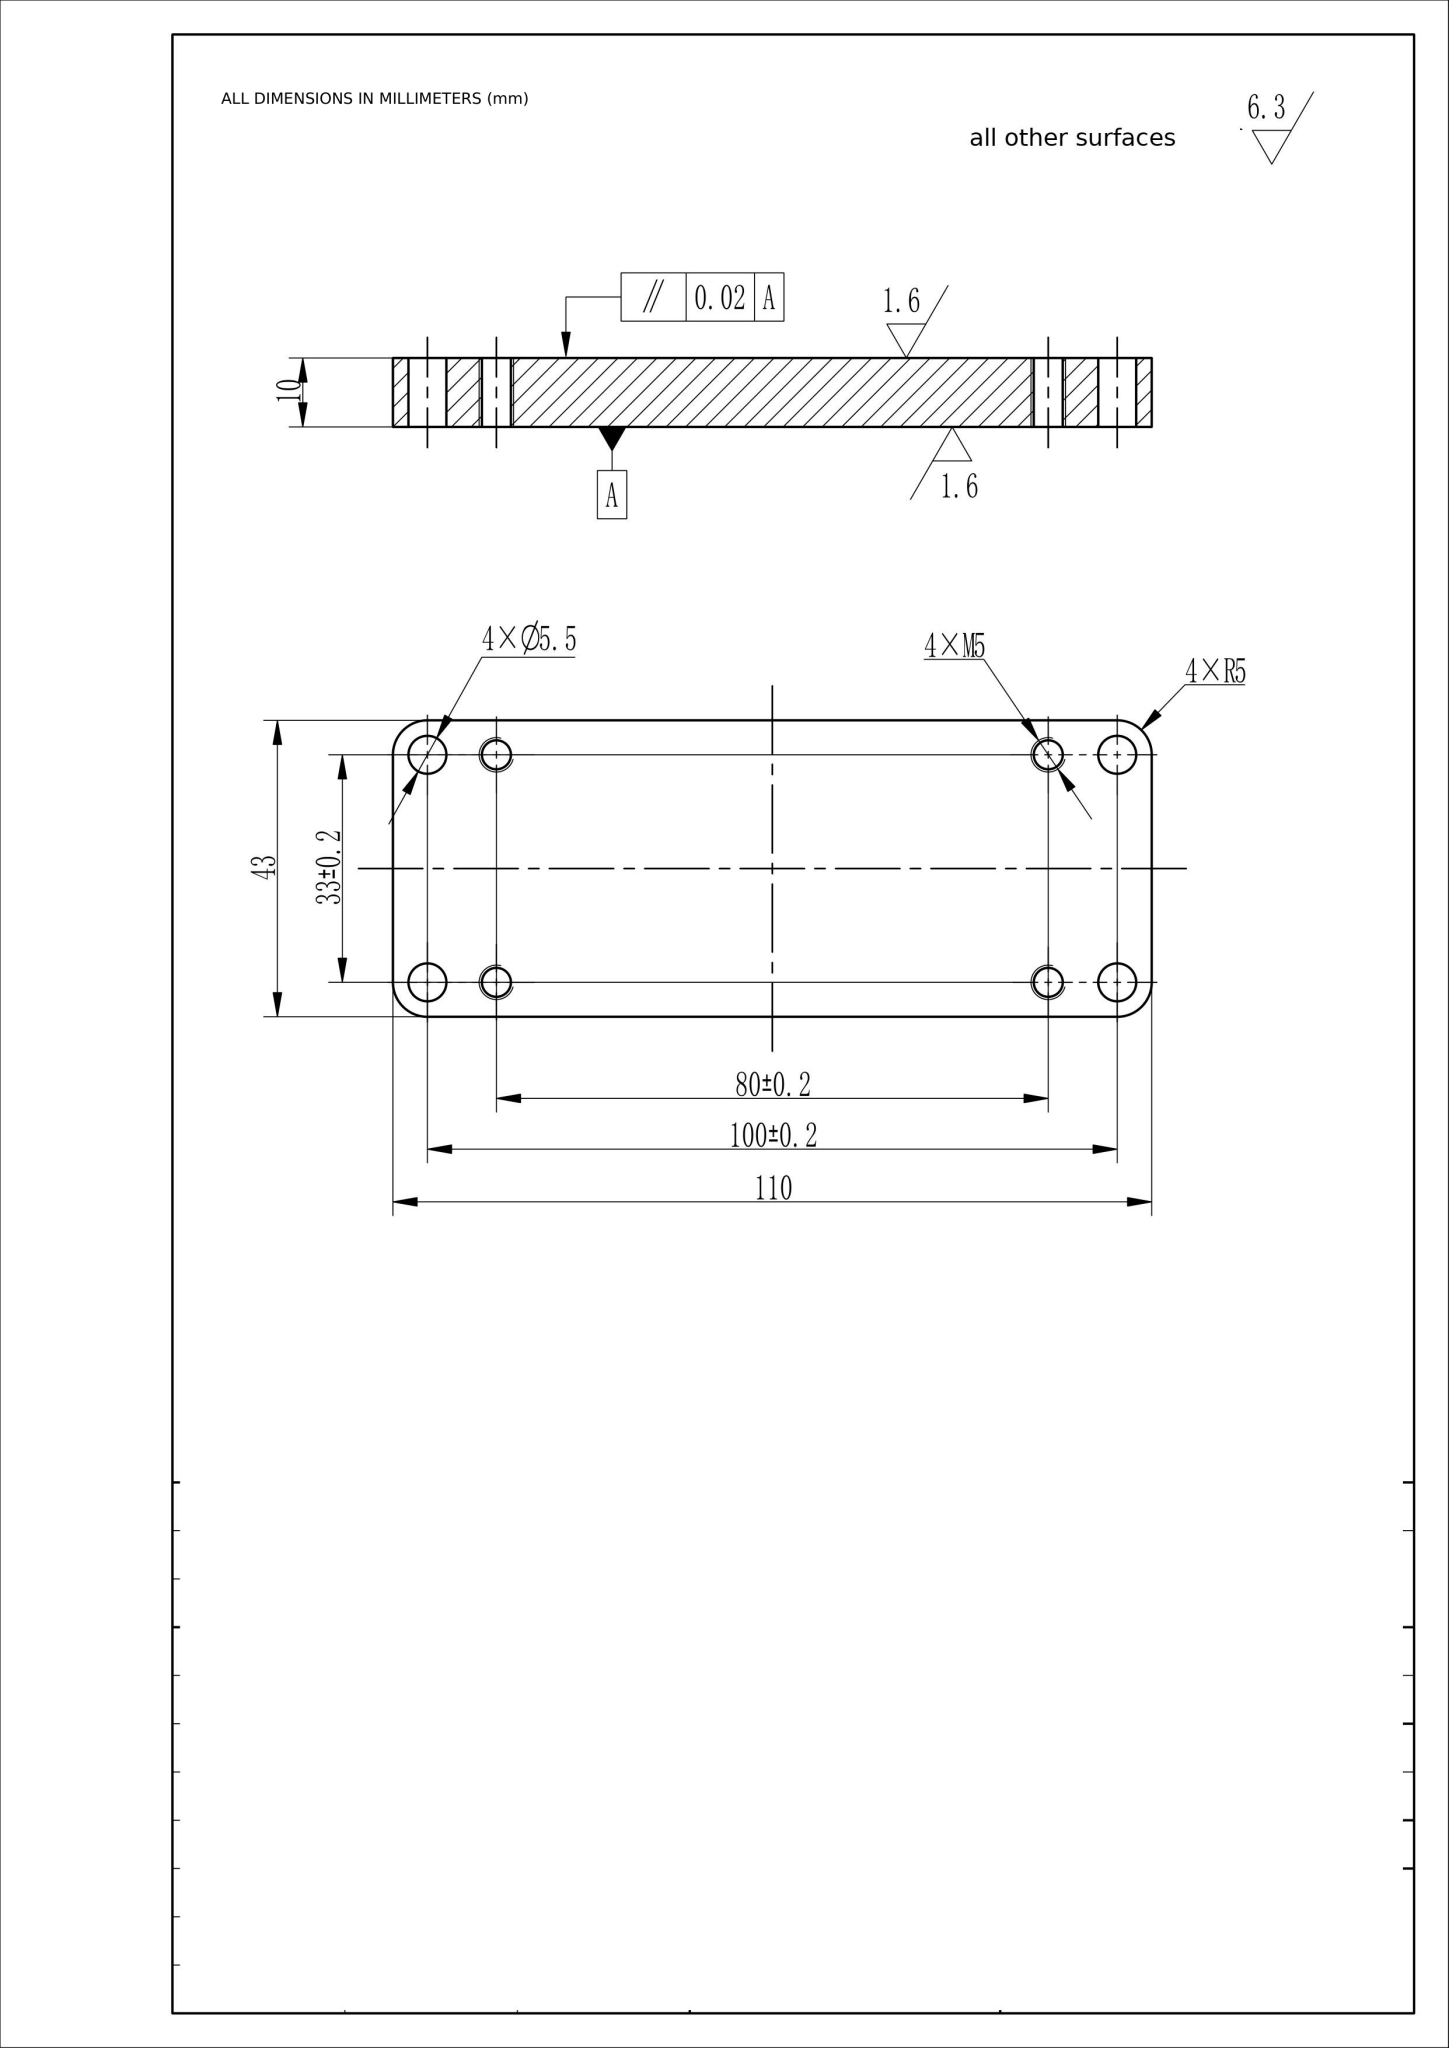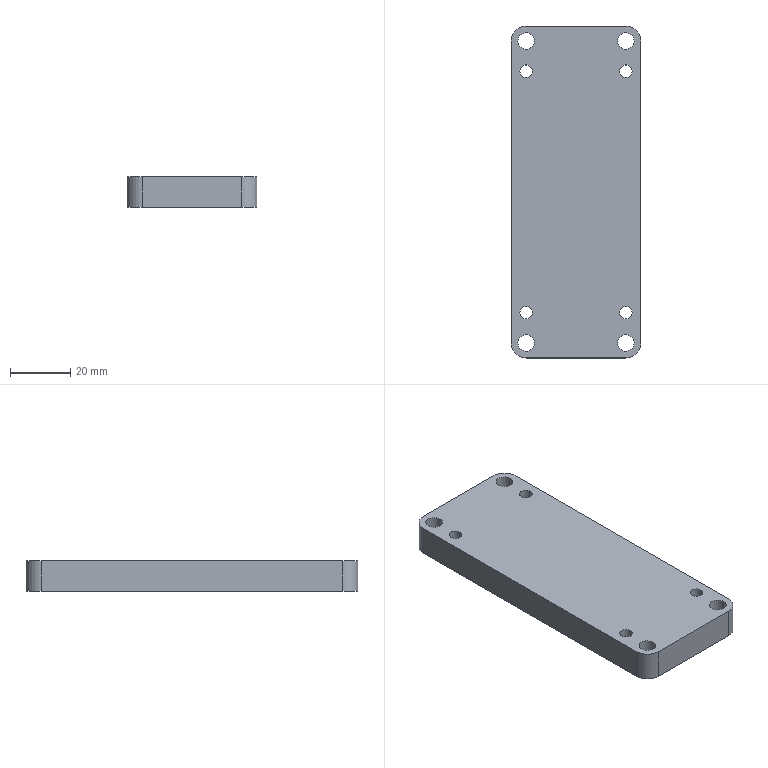Part | NX | mm | 1 solid | 18 faces | box 43 x 110 x 10 mm | volume 45581 mm3 | cylinder 12 | plane 6 | commonest cylinder face diameters 10 x4 4.2 x4 5.5 x4
STEP:
#1=CARTESIAN_POINT('',(0.,0.,0.));
#2=DIRECTION('',(0.,0.,1.));
#3=DIRECTION('',(1.,0.,0.));
#4=AXIS2_PLACEMENT_3D('',#1,#2,#3);
#5=(LENGTH_UNIT()NAMED_UNIT(*)SI_UNIT(.MILLI.,.METRE.));
#6=UNCERTAINTY_MEASURE_WITH_UNIT(LENGTH_MEASURE(0.00002),#5,'','');
#7=(NAMED_UNIT(*)PLANE_ANGLE_UNIT()SI_UNIT($,.RADIAN.));
#8=PLANE_ANGLE_MEASURE_WITH_UNIT(PLANE_ANGLE_MEASURE(0.01745),#7);
#9=DIMENSIONAL_EXPONENTS(0.,0.,0.,0.,0.,0.,0.);
#10=(CONVERSION_BASED_UNIT('',#8)NAMED_UNIT(#9)PLANE_ANGLE_UNIT());
#11=(NAMED_UNIT(*)SI_UNIT($,.STERADIAN.)SOLID_ANGLE_UNIT());
#12=(GEOMETRIC_REPRESENTATION_CONTEXT(3)GLOBAL_UNCERTAINTY_ASSIGNED_CONTEXT((#6))GLOBAL_UNIT_ASSIGNED_CONTEXT((#5,#10,#11))REPRESENTATION_CONTEXT('',''));
#13=SHAPE_REPRESENTATION('',(#4),#12);
#14=CARTESIAN_POINT('',(-21.5,50.,0.));
#15=VERTEX_POINT('',#14);
#16=CARTESIAN_POINT('',(-21.5,-50.,0.));
#17=VERTEX_POINT('',#16);
#18=CARTESIAN_POINT('',(-21.5,55.,0.));
#19=DIRECTION('',(0.,-1.,0.));
#20=VECTOR('',#19,1.);
#21=LINE('',#18,#20);
#22=EDGE_CURVE('',#15,#17,#21,.T.);
#23=ORIENTED_EDGE('',*,*,#22,.T.);
#24=CARTESIAN_POINT('',(-21.5,-50.,10.));
#25=VERTEX_POINT('',#24);
#26=CARTESIAN_POINT('',(-21.5,-50.,10.));
#27=DIRECTION('',(0.,0.,1.));
#28=VECTOR('',#27,1.);
#29=LINE('',#26,#28);
#30=EDGE_CURVE('',#17,#25,#29,.T.);
#31=ORIENTED_EDGE('',*,*,#30,.T.);
#32=CARTESIAN_POINT('',(-21.5,50.,10.));
#33=VERTEX_POINT('',#32);
#34=CARTESIAN_POINT('',(-21.5,55.,10.));
#35=DIRECTION('',(0.,-1.,0.));
#36=VECTOR('',#35,1.);
#37=LINE('',#34,#36);
#38=EDGE_CURVE('',#33,#25,#37,.T.);
#39=ORIENTED_EDGE('',*,*,#38,.F.);
#40=CARTESIAN_POINT('',(-21.5,50.,10.));
#41=DIRECTION('',(0.,0.,-1.));
#42=VECTOR('',#41,1.);
#43=LINE('',#40,#42);
#44=EDGE_CURVE('',#33,#15,#43,.T.);
#45=ORIENTED_EDGE('',*,*,#44,.T.);
#46=EDGE_LOOP('',(#23,#31,#39,#45));
#47=FACE_OUTER_BOUND('',#46,.T.);
#48=CARTESIAN_POINT('',(-21.5,55.,10.));
#49=DIRECTION('',(1.,0.,0.));
#50=DIRECTION('',(-0.,1.,0.));
#51=AXIS2_PLACEMENT_3D('',#48,#49,#50);
#52=PLANE('',#51);
#53=ADVANCED_FACE('',(#47),#52,.F.);
#54=CARTESIAN_POINT('',(-16.5,-55.,10.));
#55=VERTEX_POINT('',#54);
#56=CARTESIAN_POINT('',(16.5,-55.,10.));
#57=VERTEX_POINT('',#56);
#58=CARTESIAN_POINT('',(-21.5,-55.,10.));
#59=DIRECTION('',(1.,0.,0.));
#60=VECTOR('',#59,1.);
#61=LINE('',#58,#60);
#62=EDGE_CURVE('',#55,#57,#61,.T.);
#63=ORIENTED_EDGE('',*,*,#62,.F.);
#64=CARTESIAN_POINT('',(-16.5,-55.,0.));
#65=VERTEX_POINT('',#64);
#66=CARTESIAN_POINT('',(-16.5,-55.,10.));
#67=DIRECTION('',(0.,0.,-1.));
#68=VECTOR('',#67,1.);
#69=LINE('',#66,#68);
#70=EDGE_CURVE('',#55,#65,#69,.T.);
#71=ORIENTED_EDGE('',*,*,#70,.T.);
#72=CARTESIAN_POINT('',(16.5,-55.,0.));
#73=VERTEX_POINT('',#72);
#74=CARTESIAN_POINT('',(-21.5,-55.,0.));
#75=DIRECTION('',(1.,0.,0.));
#76=VECTOR('',#75,1.);
#77=LINE('',#74,#76);
#78=EDGE_CURVE('',#65,#73,#77,.T.);
#79=ORIENTED_EDGE('',*,*,#78,.T.);
#80=CARTESIAN_POINT('',(16.5,-55.,10.));
#81=DIRECTION('',(0.,0.,1.));
#82=VECTOR('',#81,1.);
#83=LINE('',#80,#82);
#84=EDGE_CURVE('',#73,#57,#83,.T.);
#85=ORIENTED_EDGE('',*,*,#84,.T.);
#86=EDGE_LOOP('',(#63,#71,#79,#85));
#87=FACE_OUTER_BOUND('',#86,.T.);
#88=CARTESIAN_POINT('',(-21.5,-55.,10.));
#89=DIRECTION('',(0.,1.,0.));
#90=DIRECTION('',(0.,0.,1.));
#91=AXIS2_PLACEMENT_3D('',#88,#89,#90);
#92=PLANE('',#91);
#93=ADVANCED_FACE('',(#87),#92,.F.);
#94=CARTESIAN_POINT('',(21.5,-50.,0.));
#95=VERTEX_POINT('',#94);
#96=CARTESIAN_POINT('',(21.5,50.,0.));
#97=VERTEX_POINT('',#96);
#98=CARTESIAN_POINT('',(21.5,-55.,0.));
#99=DIRECTION('',(0.,1.,0.));
#100=VECTOR('',#99,1.);
#101=LINE('',#98,#100);
#102=EDGE_CURVE('',#95,#97,#101,.T.);
#103=ORIENTED_EDGE('',*,*,#102,.T.);
#104=CARTESIAN_POINT('',(21.5,50.,10.));
#105=VERTEX_POINT('',#104);
#106=CARTESIAN_POINT('',(21.5,50.,10.));
#107=DIRECTION('',(0.,0.,1.));
#108=VECTOR('',#107,1.);
#109=LINE('',#106,#108);
#110=EDGE_CURVE('',#97,#105,#109,.T.);
#111=ORIENTED_EDGE('',*,*,#110,.T.);
#112=CARTESIAN_POINT('',(21.5,-50.,10.));
#113=VERTEX_POINT('',#112);
#114=CARTESIAN_POINT('',(21.5,-55.,10.));
#115=DIRECTION('',(0.,1.,0.));
#116=VECTOR('',#115,1.);
#117=LINE('',#114,#116);
#118=EDGE_CURVE('',#113,#105,#117,.T.);
#119=ORIENTED_EDGE('',*,*,#118,.F.);
#120=CARTESIAN_POINT('',(21.5,-50.,10.));
#121=DIRECTION('',(0.,0.,-1.));
#122=VECTOR('',#121,1.);
#123=LINE('',#120,#122);
#124=EDGE_CURVE('',#113,#95,#123,.T.);
#125=ORIENTED_EDGE('',*,*,#124,.T.);
#126=EDGE_LOOP('',(#103,#111,#119,#125));
#127=FACE_OUTER_BOUND('',#126,.T.);
#128=CARTESIAN_POINT('',(21.5,-55.,10.));
#129=DIRECTION('',(-1.,0.,0.));
#130=DIRECTION('',(0.,0.,1.));
#131=AXIS2_PLACEMENT_3D('',#128,#129,#130);
#132=PLANE('',#131);
#133=ADVANCED_FACE('',(#127),#132,.F.);
#134=CARTESIAN_POINT('',(16.5,55.,0.));
#135=VERTEX_POINT('',#134);
#136=CARTESIAN_POINT('',(-16.5,55.,0.));
#137=VERTEX_POINT('',#136);
#138=CARTESIAN_POINT('',(21.5,55.,0.));
#139=DIRECTION('',(-1.,-0.,0.));
#140=VECTOR('',#139,1.);
#141=LINE('',#138,#140);
#142=EDGE_CURVE('',#135,#137,#141,.T.);
#143=ORIENTED_EDGE('',*,*,#142,.T.);
#144=CARTESIAN_POINT('',(-16.5,55.,10.));
#145=VERTEX_POINT('',#144);
#146=CARTESIAN_POINT('',(-16.5,55.,10.));
#147=DIRECTION('',(0.,0.,1.));
#148=VECTOR('',#147,1.);
#149=LINE('',#146,#148);
#150=EDGE_CURVE('',#137,#145,#149,.T.);
#151=ORIENTED_EDGE('',*,*,#150,.T.);
#152=CARTESIAN_POINT('',(16.5,55.,10.));
#153=VERTEX_POINT('',#152);
#154=CARTESIAN_POINT('',(21.5,55.,10.));
#155=DIRECTION('',(-1.,-0.,0.));
#156=VECTOR('',#155,1.);
#157=LINE('',#154,#156);
#158=EDGE_CURVE('',#153,#145,#157,.T.);
#159=ORIENTED_EDGE('',*,*,#158,.F.);
#160=CARTESIAN_POINT('',(16.5,55.,10.));
#161=DIRECTION('',(0.,0.,-1.));
#162=VECTOR('',#161,1.);
#163=LINE('',#160,#162);
#164=EDGE_CURVE('',#153,#135,#163,.T.);
#165=ORIENTED_EDGE('',*,*,#164,.T.);
#166=EDGE_LOOP('',(#143,#151,#159,#165));
#167=FACE_OUTER_BOUND('',#166,.T.);
#168=CARTESIAN_POINT('',(21.5,55.,10.));
#169=DIRECTION('',(0.,-1.,0.));
#170=DIRECTION('',(1.,0.,0.));
#171=AXIS2_PLACEMENT_3D('',#168,#169,#170);
#172=PLANE('',#171);
#173=ADVANCED_FACE('',(#167),#172,.F.);
#174=CARTESIAN_POINT('',(13.75,50.,10.));
#175=VERTEX_POINT('',#174);
#176=CARTESIAN_POINT('',(16.5,50.,10.));
#177=DIRECTION('',(0.,0.,-1.));
#178=DIRECTION('',(-1.,0.,0.));
#179=AXIS2_PLACEMENT_3D('',#176,#177,#178);
#180=CIRCLE('',#179,2.75);
#181=EDGE_CURVE('',#175,#175,#180,.T.);
#182=ORIENTED_EDGE('',*,*,#181,.T.);
#183=EDGE_LOOP('',(#182));
#184=FACE_BOUND('',#183,.T.);
#185=CARTESIAN_POINT('',(13.75,-50.,10.));
#186=VERTEX_POINT('',#185);
#187=CARTESIAN_POINT('',(16.5,-50.,10.));
#188=DIRECTION('',(0.,0.,-1.));
#189=DIRECTION('',(-1.,0.,0.));
#190=AXIS2_PLACEMENT_3D('',#187,#188,#189);
#191=CIRCLE('',#190,2.75);
#192=EDGE_CURVE('',#186,#186,#191,.T.);
#193=ORIENTED_EDGE('',*,*,#192,.T.);
#194=EDGE_LOOP('',(#193));
#195=FACE_BOUND('',#194,.T.);
#196=CARTESIAN_POINT('',(-19.25,50.,10.));
#197=VERTEX_POINT('',#196);
#198=CARTESIAN_POINT('',(-16.5,50.,10.));
#199=DIRECTION('',(0.,0.,-1.));
#200=DIRECTION('',(-1.,0.,0.));
#201=AXIS2_PLACEMENT_3D('',#198,#199,#200);
#202=CIRCLE('',#201,2.75);
#203=EDGE_CURVE('',#197,#197,#202,.T.);
#204=ORIENTED_EDGE('',*,*,#203,.T.);
#205=EDGE_LOOP('',(#204));
#206=FACE_BOUND('',#205,.T.);
#207=CARTESIAN_POINT('',(-19.25,-50.,10.));
#208=VERTEX_POINT('',#207);
#209=CARTESIAN_POINT('',(-16.5,-50.,10.));
#210=DIRECTION('',(0.,0.,-1.));
#211=DIRECTION('',(-1.,0.,0.));
#212=AXIS2_PLACEMENT_3D('',#209,#210,#211);
#213=CIRCLE('',#212,2.75);
#214=EDGE_CURVE('',#208,#208,#213,.T.);
#215=ORIENTED_EDGE('',*,*,#214,.T.);
#216=EDGE_LOOP('',(#215));
#217=FACE_BOUND('',#216,.T.);
#218=CARTESIAN_POINT('',(14.4,40.,10.));
#219=VERTEX_POINT('',#218);
#220=CARTESIAN_POINT('',(16.5,40.,10.));
#221=DIRECTION('',(0.,0.,-1.));
#222=DIRECTION('',(-1.,0.,0.));
#223=AXIS2_PLACEMENT_3D('',#220,#221,#222);
#224=CIRCLE('',#223,2.1);
#225=EDGE_CURVE('',#219,#219,#224,.T.);
#226=ORIENTED_EDGE('',*,*,#225,.T.);
#227=EDGE_LOOP('',(#226));
#228=FACE_BOUND('',#227,.T.);
#229=CARTESIAN_POINT('',(14.4,-40.,10.));
#230=VERTEX_POINT('',#229);
#231=CARTESIAN_POINT('',(16.5,-40.,10.));
#232=DIRECTION('',(0.,0.,-1.));
#233=DIRECTION('',(-1.,0.,0.));
#234=AXIS2_PLACEMENT_3D('',#231,#232,#233);
#235=CIRCLE('',#234,2.1);
#236=EDGE_CURVE('',#230,#230,#235,.T.);
#237=ORIENTED_EDGE('',*,*,#236,.T.);
#238=EDGE_LOOP('',(#237));
#239=FACE_BOUND('',#238,.T.);
#240=CARTESIAN_POINT('',(-18.6,40.,10.));
#241=VERTEX_POINT('',#240);
#242=CARTESIAN_POINT('',(-16.5,40.,10.));
#243=DIRECTION('',(0.,0.,-1.));
#244=DIRECTION('',(-1.,0.,0.));
#245=AXIS2_PLACEMENT_3D('',#242,#243,#244);
#246=CIRCLE('',#245,2.1);
#247=EDGE_CURVE('',#241,#241,#246,.T.);
#248=ORIENTED_EDGE('',*,*,#247,.T.);
#249=EDGE_LOOP('',(#248));
#250=FACE_BOUND('',#249,.T.);
#251=CARTESIAN_POINT('',(-18.6,-40.,10.));
#252=VERTEX_POINT('',#251);
#253=CARTESIAN_POINT('',(-16.5,-40.,10.));
#254=DIRECTION('',(0.,0.,-1.));
#255=DIRECTION('',(-1.,0.,0.));
#256=AXIS2_PLACEMENT_3D('',#253,#254,#255);
#257=CIRCLE('',#256,2.1);
#258=EDGE_CURVE('',#252,#252,#257,.T.);
#259=ORIENTED_EDGE('',*,*,#258,.T.);
#260=EDGE_LOOP('',(#259));
#261=FACE_BOUND('',#260,.T.);
#262=ORIENTED_EDGE('',*,*,#38,.T.);
#263=CARTESIAN_POINT('',(-16.5,-50.,10.));
#264=DIRECTION('',(0.,0.,1.));
#265=DIRECTION('',(1.,0.,0.));
#266=AXIS2_PLACEMENT_3D('',#263,#264,#265);
#267=CIRCLE('',#266,5.);
#268=EDGE_CURVE('',#25,#55,#267,.T.);
#269=ORIENTED_EDGE('',*,*,#268,.T.);
#270=ORIENTED_EDGE('',*,*,#62,.T.);
#271=CARTESIAN_POINT('',(16.5,-50.,10.));
#272=DIRECTION('',(0.,0.,1.));
#273=DIRECTION('',(1.,0.,0.));
#274=AXIS2_PLACEMENT_3D('',#271,#272,#273);
#275=CIRCLE('',#274,5.);
#276=EDGE_CURVE('',#57,#113,#275,.T.);
#277=ORIENTED_EDGE('',*,*,#276,.T.);
#278=ORIENTED_EDGE('',*,*,#118,.T.);
#279=CARTESIAN_POINT('',(16.5,50.,10.));
#280=DIRECTION('',(0.,0.,1.));
#281=DIRECTION('',(1.,0.,0.));
#282=AXIS2_PLACEMENT_3D('',#279,#280,#281);
#283=CIRCLE('',#282,5.);
#284=EDGE_CURVE('',#105,#153,#283,.T.);
#285=ORIENTED_EDGE('',*,*,#284,.T.);
#286=ORIENTED_EDGE('',*,*,#158,.T.);
#287=CARTESIAN_POINT('',(-16.5,50.,10.));
#288=DIRECTION('',(0.,0.,1.));
#289=DIRECTION('',(1.,0.,0.));
#290=AXIS2_PLACEMENT_3D('',#287,#288,#289);
#291=CIRCLE('',#290,5.);
#292=EDGE_CURVE('',#145,#33,#291,.T.);
#293=ORIENTED_EDGE('',*,*,#292,.T.);
#294=EDGE_LOOP('',(#262,#269,#270,#277,#278,#285,#286,#293));
#295=FACE_BOUND('',#294,.T.);
#296=CARTESIAN_POINT('',(0.,0.,10.));
#297=DIRECTION('',(0.,0.,1.));
#298=DIRECTION('',(1.,0.,0.));
#299=AXIS2_PLACEMENT_3D('',#296,#297,#298);
#300=PLANE('',#299);
#301=ADVANCED_FACE('',(#184,#195,#206,#217,#228,#239,#250,#261,#295),#300,.T.);
#302=CARTESIAN_POINT('',(13.75,50.,0.));
#303=VERTEX_POINT('',#302);
#304=CARTESIAN_POINT('',(16.5,50.,0.));
#305=DIRECTION('',(0.,0.,-1.));
#306=DIRECTION('',(-1.,0.,0.));
#307=AXIS2_PLACEMENT_3D('',#304,#305,#306);
#308=CIRCLE('',#307,2.75);
#309=EDGE_CURVE('',#303,#303,#308,.T.);
#310=ORIENTED_EDGE('',*,*,#309,.F.);
#311=EDGE_LOOP('',(#310));
#312=FACE_BOUND('',#311,.T.);
#313=CARTESIAN_POINT('',(13.75,-50.,0.));
#314=VERTEX_POINT('',#313);
#315=CARTESIAN_POINT('',(16.5,-50.,0.));
#316=DIRECTION('',(0.,0.,-1.));
#317=DIRECTION('',(-1.,0.,0.));
#318=AXIS2_PLACEMENT_3D('',#315,#316,#317);
#319=CIRCLE('',#318,2.75);
#320=EDGE_CURVE('',#314,#314,#319,.T.);
#321=ORIENTED_EDGE('',*,*,#320,.F.);
#322=EDGE_LOOP('',(#321));
#323=FACE_BOUND('',#322,.T.);
#324=CARTESIAN_POINT('',(-19.25,50.,0.));
#325=VERTEX_POINT('',#324);
#326=CARTESIAN_POINT('',(-16.5,50.,0.));
#327=DIRECTION('',(0.,0.,-1.));
#328=DIRECTION('',(-1.,0.,0.));
#329=AXIS2_PLACEMENT_3D('',#326,#327,#328);
#330=CIRCLE('',#329,2.75);
#331=EDGE_CURVE('',#325,#325,#330,.T.);
#332=ORIENTED_EDGE('',*,*,#331,.F.);
#333=EDGE_LOOP('',(#332));
#334=FACE_BOUND('',#333,.T.);
#335=CARTESIAN_POINT('',(-19.25,-50.,0.));
#336=VERTEX_POINT('',#335);
#337=CARTESIAN_POINT('',(-16.5,-50.,0.));
#338=DIRECTION('',(0.,0.,-1.));
#339=DIRECTION('',(-1.,0.,0.));
#340=AXIS2_PLACEMENT_3D('',#337,#338,#339);
#341=CIRCLE('',#340,2.75);
#342=EDGE_CURVE('',#336,#336,#341,.T.);
#343=ORIENTED_EDGE('',*,*,#342,.F.);
#344=EDGE_LOOP('',(#343));
#345=FACE_BOUND('',#344,.T.);
#346=CARTESIAN_POINT('',(14.4,40.,0.));
#347=VERTEX_POINT('',#346);
#348=CARTESIAN_POINT('',(16.5,40.,0.));
#349=DIRECTION('',(0.,0.,-1.));
#350=DIRECTION('',(-1.,0.,0.));
#351=AXIS2_PLACEMENT_3D('',#348,#349,#350);
#352=CIRCLE('',#351,2.1);
#353=EDGE_CURVE('',#347,#347,#352,.T.);
#354=ORIENTED_EDGE('',*,*,#353,.F.);
#355=EDGE_LOOP('',(#354));
#356=FACE_BOUND('',#355,.T.);
#357=CARTESIAN_POINT('',(14.4,-40.,0.));
#358=VERTEX_POINT('',#357);
#359=CARTESIAN_POINT('',(16.5,-40.,0.));
#360=DIRECTION('',(0.,0.,-1.));
#361=DIRECTION('',(-1.,0.,0.));
#362=AXIS2_PLACEMENT_3D('',#359,#360,#361);
#363=CIRCLE('',#362,2.1);
#364=EDGE_CURVE('',#358,#358,#363,.T.);
#365=ORIENTED_EDGE('',*,*,#364,.F.);
#366=EDGE_LOOP('',(#365));
#367=FACE_BOUND('',#366,.T.);
#368=CARTESIAN_POINT('',(-18.6,40.,0.));
#369=VERTEX_POINT('',#368);
#370=CARTESIAN_POINT('',(-16.5,40.,0.));
#371=DIRECTION('',(0.,0.,-1.));
#372=DIRECTION('',(-1.,0.,0.));
#373=AXIS2_PLACEMENT_3D('',#370,#371,#372);
#374=CIRCLE('',#373,2.1);
#375=EDGE_CURVE('',#369,#369,#374,.T.);
#376=ORIENTED_EDGE('',*,*,#375,.F.);
#377=EDGE_LOOP('',(#376));
#378=FACE_BOUND('',#377,.T.);
#379=CARTESIAN_POINT('',(-18.6,-40.,0.));
#380=VERTEX_POINT('',#379);
#381=CARTESIAN_POINT('',(-16.5,-40.,0.));
#382=DIRECTION('',(0.,0.,-1.));
#383=DIRECTION('',(-1.,0.,0.));
#384=AXIS2_PLACEMENT_3D('',#381,#382,#383);
#385=CIRCLE('',#384,2.1);
#386=EDGE_CURVE('',#380,#380,#385,.T.);
#387=ORIENTED_EDGE('',*,*,#386,.F.);
#388=EDGE_LOOP('',(#387));
#389=FACE_BOUND('',#388,.T.);
#390=ORIENTED_EDGE('',*,*,#78,.F.);
#391=CARTESIAN_POINT('',(-16.5,-50.,0.));
#392=DIRECTION('',(0.,0.,-1.));
#393=DIRECTION('',(1.,0.,0.));
#394=AXIS2_PLACEMENT_3D('',#391,#392,#393);
#395=CIRCLE('',#394,5.);
#396=EDGE_CURVE('',#65,#17,#395,.T.);
#397=ORIENTED_EDGE('',*,*,#396,.T.);
#398=ORIENTED_EDGE('',*,*,#22,.F.);
#399=CARTESIAN_POINT('',(-16.5,50.,0.));
#400=DIRECTION('',(0.,0.,-1.));
#401=DIRECTION('',(1.,0.,0.));
#402=AXIS2_PLACEMENT_3D('',#399,#400,#401);
#403=CIRCLE('',#402,5.);
#404=EDGE_CURVE('',#15,#137,#403,.T.);
#405=ORIENTED_EDGE('',*,*,#404,.T.);
#406=ORIENTED_EDGE('',*,*,#142,.F.);
#407=CARTESIAN_POINT('',(16.5,50.,0.));
#408=DIRECTION('',(0.,0.,-1.));
#409=DIRECTION('',(1.,0.,0.));
#410=AXIS2_PLACEMENT_3D('',#407,#408,#409);
#411=CIRCLE('',#410,5.);
#412=EDGE_CURVE('',#135,#97,#411,.T.);
#413=ORIENTED_EDGE('',*,*,#412,.T.);
#414=ORIENTED_EDGE('',*,*,#102,.F.);
#415=CARTESIAN_POINT('',(16.5,-50.,0.));
#416=DIRECTION('',(0.,0.,-1.));
#417=DIRECTION('',(1.,0.,0.));
#418=AXIS2_PLACEMENT_3D('',#415,#416,#417);
#419=CIRCLE('',#418,5.);
#420=EDGE_CURVE('',#95,#73,#419,.T.);
#421=ORIENTED_EDGE('',*,*,#420,.T.);
#422=EDGE_LOOP('',(#390,#397,#398,#405,#406,#413,#414,#421));
#423=FACE_BOUND('',#422,.T.);
#424=CARTESIAN_POINT('',(0.,0.,0.));
#425=DIRECTION('',(0.,0.,1.));
#426=DIRECTION('',(1.,0.,0.));
#427=AXIS2_PLACEMENT_3D('',#424,#425,#426);
#428=PLANE('',#427);
#429=ADVANCED_FACE('',(#312,#323,#334,#345,#356,#367,#378,#389,#423),#428,.F.);
#430=ORIENTED_EDGE('',*,*,#268,.F.);
#431=ORIENTED_EDGE('',*,*,#30,.F.);
#432=ORIENTED_EDGE('',*,*,#396,.F.);
#433=ORIENTED_EDGE('',*,*,#70,.F.);
#434=EDGE_LOOP('',(#430,#431,#432,#433));
#435=FACE_OUTER_BOUND('',#434,.T.);
#436=CARTESIAN_POINT('',(-16.5,-50.,10.));
#437=DIRECTION('',(0.,0.,-1.));
#438=DIRECTION('',(-1.,0.,0.));
#439=AXIS2_PLACEMENT_3D('',#436,#437,#438);
#440=CYLINDRICAL_SURFACE('',#439,5.);
#441=ADVANCED_FACE('',(#435),#440,.T.);
#442=ORIENTED_EDGE('',*,*,#292,.F.);
#443=ORIENTED_EDGE('',*,*,#150,.F.);
#444=ORIENTED_EDGE('',*,*,#404,.F.);
#445=ORIENTED_EDGE('',*,*,#44,.F.);
#446=EDGE_LOOP('',(#442,#443,#444,#445));
#447=FACE_OUTER_BOUND('',#446,.T.);
#448=CARTESIAN_POINT('',(-16.5,50.,10.));
#449=DIRECTION('',(0.,0.,-1.));
#450=DIRECTION('',(-1.,0.,0.));
#451=AXIS2_PLACEMENT_3D('',#448,#449,#450);
#452=CYLINDRICAL_SURFACE('',#451,5.);
#453=ADVANCED_FACE('',(#447),#452,.T.);
#454=ORIENTED_EDGE('',*,*,#284,.F.);
#455=ORIENTED_EDGE('',*,*,#110,.F.);
#456=ORIENTED_EDGE('',*,*,#412,.F.);
#457=ORIENTED_EDGE('',*,*,#164,.F.);
#458=EDGE_LOOP('',(#454,#455,#456,#457));
#459=FACE_OUTER_BOUND('',#458,.T.);
#460=CARTESIAN_POINT('',(16.5,50.,10.));
#461=DIRECTION('',(0.,0.,-1.));
#462=DIRECTION('',(-1.,0.,0.));
#463=AXIS2_PLACEMENT_3D('',#460,#461,#462);
#464=CYLINDRICAL_SURFACE('',#463,5.);
#465=ADVANCED_FACE('',(#459),#464,.T.);
#466=ORIENTED_EDGE('',*,*,#276,.F.);
#467=ORIENTED_EDGE('',*,*,#84,.F.);
#468=ORIENTED_EDGE('',*,*,#420,.F.);
#469=ORIENTED_EDGE('',*,*,#124,.F.);
#470=EDGE_LOOP('',(#466,#467,#468,#469));
#471=FACE_OUTER_BOUND('',#470,.T.);
#472=CARTESIAN_POINT('',(16.5,-50.,10.));
#473=DIRECTION('',(0.,0.,-1.));
#474=DIRECTION('',(-1.,0.,0.));
#475=AXIS2_PLACEMENT_3D('',#472,#473,#474);
#476=CYLINDRICAL_SURFACE('',#475,5.);
#477=ADVANCED_FACE('',(#471),#476,.T.);
#478=ORIENTED_EDGE('',*,*,#386,.T.);
#479=EDGE_LOOP('',(#478));
#480=FACE_BOUND('',#479,.T.);
#481=ORIENTED_EDGE('',*,*,#258,.F.);
#482=EDGE_LOOP('',(#481));
#483=FACE_BOUND('',#482,.T.);
#484=CARTESIAN_POINT('',(-16.5,-40.,10.));
#485=DIRECTION('',(0.,0.,-1.));
#486=DIRECTION('',(-1.,0.,0.));
#487=AXIS2_PLACEMENT_3D('',#484,#485,#486);
#488=CYLINDRICAL_SURFACE('',#487,2.1);
#489=ADVANCED_FACE('',(#480,#483),#488,.F.);
#490=ORIENTED_EDGE('',*,*,#375,.T.);
#491=EDGE_LOOP('',(#490));
#492=FACE_BOUND('',#491,.T.);
#493=ORIENTED_EDGE('',*,*,#247,.F.);
#494=EDGE_LOOP('',(#493));
#495=FACE_BOUND('',#494,.T.);
#496=CARTESIAN_POINT('',(-16.5,40.,10.));
#497=DIRECTION('',(0.,0.,-1.));
#498=DIRECTION('',(-1.,0.,0.));
#499=AXIS2_PLACEMENT_3D('',#496,#497,#498);
#500=CYLINDRICAL_SURFACE('',#499,2.1);
#501=ADVANCED_FACE('',(#492,#495),#500,.F.);
#502=ORIENTED_EDGE('',*,*,#364,.T.);
#503=EDGE_LOOP('',(#502));
#504=FACE_BOUND('',#503,.T.);
#505=ORIENTED_EDGE('',*,*,#236,.F.);
#506=EDGE_LOOP('',(#505));
#507=FACE_BOUND('',#506,.T.);
#508=CARTESIAN_POINT('',(16.5,-40.,10.));
#509=DIRECTION('',(0.,0.,-1.));
#510=DIRECTION('',(-1.,0.,0.));
#511=AXIS2_PLACEMENT_3D('',#508,#509,#510);
#512=CYLINDRICAL_SURFACE('',#511,2.1);
#513=ADVANCED_FACE('',(#504,#507),#512,.F.);
#514=ORIENTED_EDGE('',*,*,#353,.T.);
#515=EDGE_LOOP('',(#514));
#516=FACE_BOUND('',#515,.T.);
#517=ORIENTED_EDGE('',*,*,#225,.F.);
#518=EDGE_LOOP('',(#517));
#519=FACE_BOUND('',#518,.T.);
#520=CARTESIAN_POINT('',(16.5,40.,10.));
#521=DIRECTION('',(0.,0.,-1.));
#522=DIRECTION('',(-1.,0.,0.));
#523=AXIS2_PLACEMENT_3D('',#520,#521,#522);
#524=CYLINDRICAL_SURFACE('',#523,2.1);
#525=ADVANCED_FACE('',(#516,#519),#524,.F.);
#526=ORIENTED_EDGE('',*,*,#342,.T.);
#527=EDGE_LOOP('',(#526));
#528=FACE_BOUND('',#527,.T.);
#529=ORIENTED_EDGE('',*,*,#214,.F.);
#530=EDGE_LOOP('',(#529));
#531=FACE_BOUND('',#530,.T.);
#532=CARTESIAN_POINT('',(-16.5,-50.,10.));
#533=DIRECTION('',(0.,0.,-1.));
#534=DIRECTION('',(-1.,0.,0.));
#535=AXIS2_PLACEMENT_3D('',#532,#533,#534);
#536=CYLINDRICAL_SURFACE('',#535,2.75);
#537=ADVANCED_FACE('',(#528,#531),#536,.F.);
#538=ORIENTED_EDGE('',*,*,#331,.T.);
#539=EDGE_LOOP('',(#538));
#540=FACE_BOUND('',#539,.T.);
#541=ORIENTED_EDGE('',*,*,#203,.F.);
#542=EDGE_LOOP('',(#541));
#543=FACE_BOUND('',#542,.T.);
#544=CARTESIAN_POINT('',(-16.5,50.,10.));
#545=DIRECTION('',(0.,0.,-1.));
#546=DIRECTION('',(-1.,0.,0.));
#547=AXIS2_PLACEMENT_3D('',#544,#545,#546);
#548=CYLINDRICAL_SURFACE('',#547,2.75);
#549=ADVANCED_FACE('',(#540,#543),#548,.F.);
#550=ORIENTED_EDGE('',*,*,#320,.T.);
#551=EDGE_LOOP('',(#550));
#552=FACE_BOUND('',#551,.T.);
#553=ORIENTED_EDGE('',*,*,#192,.F.);
#554=EDGE_LOOP('',(#553));
#555=FACE_BOUND('',#554,.T.);
#556=CARTESIAN_POINT('',(16.5,-50.,10.));
#557=DIRECTION('',(0.,0.,-1.));
#558=DIRECTION('',(-1.,0.,0.));
#559=AXIS2_PLACEMENT_3D('',#556,#557,#558);
#560=CYLINDRICAL_SURFACE('',#559,2.75);
#561=ADVANCED_FACE('',(#552,#555),#560,.F.);
#562=ORIENTED_EDGE('',*,*,#309,.T.);
#563=EDGE_LOOP('',(#562));
#564=FACE_BOUND('',#563,.T.);
#565=ORIENTED_EDGE('',*,*,#181,.F.);
#566=EDGE_LOOP('',(#565));
#567=FACE_BOUND('',#566,.T.);
#568=CARTESIAN_POINT('',(16.5,50.,10.));
#569=DIRECTION('',(0.,0.,-1.));
#570=DIRECTION('',(-1.,0.,0.));
#571=AXIS2_PLACEMENT_3D('',#568,#569,#570);
#572=CYLINDRICAL_SURFACE('',#571,2.75);
#573=ADVANCED_FACE('',(#564,#567),#572,.F.);
#574=CLOSED_SHELL('',(#53,#93,#133,#173,#301,#429,#441,#453,#465,#477,#489,#501,#513,#525,#537,#549,#561,#573));
#575=MANIFOLD_SOLID_BREP('',#574);
#576=ADVANCED_BREP_SHAPE_REPRESENTATION('',(#575),#12);
#577=SHAPE_REPRESENTATION_RELATIONSHIP('','',#13,#576);
#578=PRESENTATION_LAYER_ASSIGNMENT('','',(#575));
#579=COLOUR_RGB('',0.8,0.6,0.);
#580=FILL_AREA_STYLE_COLOUR('',#579);
#581=FILL_AREA_STYLE('',(#580));
#582=SURFACE_STYLE_FILL_AREA(#581);
#583=SURFACE_SIDE_STYLE('',(#582));
#584=SURFACE_STYLE_USAGE(.BOTH.,#583);
#585=PRESENTATION_STYLE_ASSIGNMENT((#584));
#586=STYLED_ITEM('',(#585),#575);
#587=MECHANICAL_DESIGN_GEOMETRIC_PRESENTATION_REPRESENTATION('',(#586),#12);